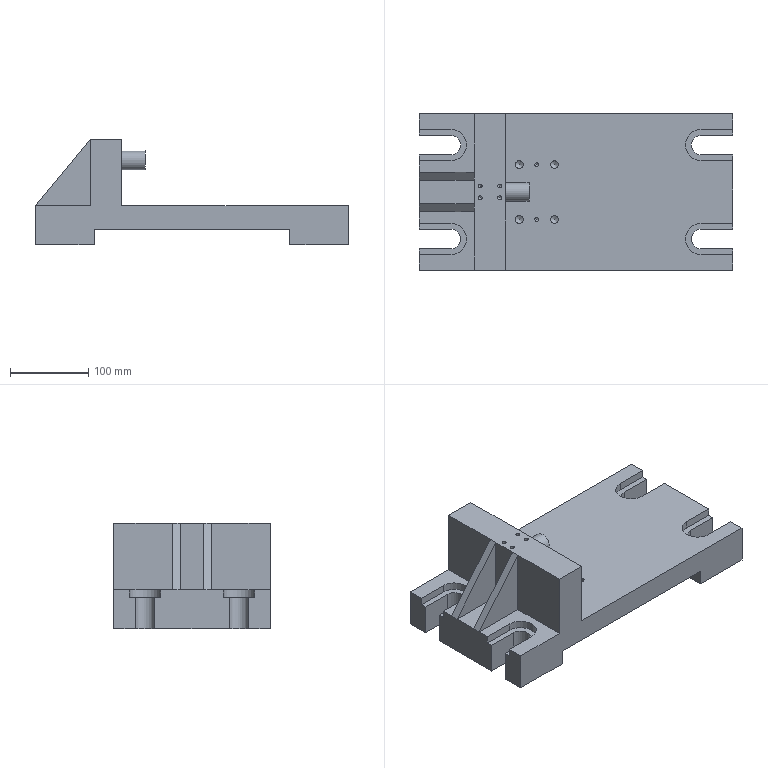Component | NX | FIXTURE_BODY | 1 solid | 80 faces | volume 3452465 mm3 | plane 49 | cylinder 20 | cone 11 | commonest cylinder face diameters 5 x6 10 x5 40 x4 25 x4 24 x1